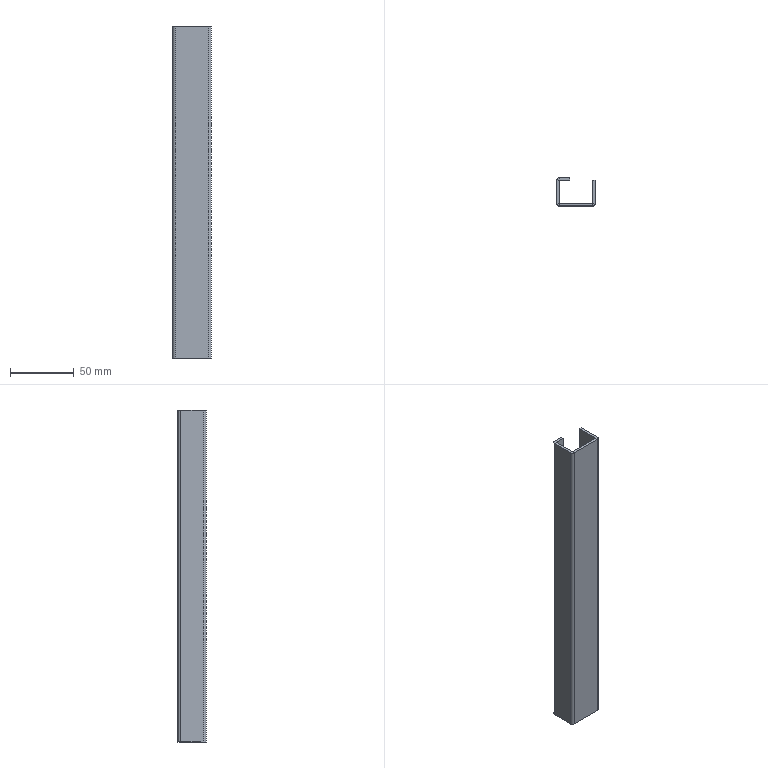Component | SolidWorks | Cover1XG1-2 | 1 solid | 30 faces | box 30 x 22 x 260 mm | volume 38817 mm3 | plane 24 | cylinder 6 | commonest cylinder face diameters 0.1 x3 4.1 x3
STEP:
#1=COLOUR_RGB('',0.7922,0.8196,0.9333);
#2=FILL_AREA_STYLE_COLOUR('',#1);
#3=FILL_AREA_STYLE('',(#2));
#4=SURFACE_STYLE_FILL_AREA(#3);
#5=SURFACE_SIDE_STYLE('',(#4));
#6=SURFACE_STYLE_USAGE(.BOTH.,#5);
#7=PRESENTATION_STYLE_ASSIGNMENT((#6));
#8=CARTESIAN_POINT('',(-5.827,-6.297,10.236));
#9=VERTEX_POINT('',#8);
#10=CARTESIAN_POINT('',(-5.827,-5.593,10.236));
#11=VERTEX_POINT('',#10);
#12=CARTESIAN_POINT('',(-5.827,-6.378,10.236));
#13=DIRECTION('',(0.,1.,0.));
#14=VECTOR('',#13,39.37);
#15=LINE('',#12,#14);
#16=EDGE_CURVE('',#9,#11,#15,.T.);
#17=ORIENTED_EDGE('',*,*,#16,.T.);
#18=CARTESIAN_POINT('',(-5.906,-5.593,10.236));
#19=VERTEX_POINT('',#18);
#20=CARTESIAN_POINT('',(-5.827,-5.593,10.236));
#21=DIRECTION('',(-1.,0.,0.));
#22=VECTOR('',#21,39.37);
#23=LINE('',#20,#22);
#24=EDGE_CURVE('',#11,#19,#23,.T.);
#25=ORIENTED_EDGE('',*,*,#24,.T.);
#26=CARTESIAN_POINT('',(-5.906,-6.297,10.236));
#27=VERTEX_POINT('',#26);
#28=CARTESIAN_POINT('',(-5.906,-6.378,10.236));
#29=DIRECTION('',(0.,1.,0.));
#30=VECTOR('',#29,39.37);
#31=LINE('',#28,#30);
#32=EDGE_CURVE('',#27,#19,#31,.T.);
#33=ORIENTED_EDGE('',*,*,#32,.F.);
#34=CARTESIAN_POINT('',(-5.906,-6.297,10.236));
#35=DIRECTION('',(1.,-0.,0.));
#36=VECTOR('',#35,39.37);
#37=LINE('',#34,#36);
#38=EDGE_CURVE('',#27,#9,#37,.T.);
#39=ORIENTED_EDGE('',*,*,#38,.T.);
#40=EDGE_LOOP('',(#17,#25,#33,#39));
#41=FACE_OUTER_BOUND('',#40,.T.);
#42=CARTESIAN_POINT('',(-5.825,-6.299,10.236));
#43=DIRECTION('',(0.,0.,1.));
#44=DIRECTION('',(-1.,0.,0.));
#45=AXIS2_PLACEMENT_3D('',#42,#43,#44);
#46=PLANE('',#45);
#47=ADVANCED_FACE('',(#41),#46,.T.);
#48=CARTESIAN_POINT('',(-5.906,-5.593,0.));
#49=VERTEX_POINT('',#48);
#50=CARTESIAN_POINT('',(-5.906,-5.593,10.236));
#51=DIRECTION('',(0.,0.,-1.));
#52=VECTOR('',#51,39.37);
#53=LINE('',#50,#52);
#54=EDGE_CURVE('',#19,#49,#53,.T.);
#55=ORIENTED_EDGE('',*,*,#54,.T.);
#56=CARTESIAN_POINT('',(-5.906,-6.297,0.));
#57=VERTEX_POINT('',#56);
#58=CARTESIAN_POINT('',(-5.906,-6.378,0.));
#59=DIRECTION('',(0.,1.,0.));
#60=VECTOR('',#59,39.37);
#61=LINE('',#58,#60);
#62=EDGE_CURVE('',#57,#49,#61,.T.);
#63=ORIENTED_EDGE('',*,*,#62,.F.);
#64=CARTESIAN_POINT('',(-5.906,-6.297,0.));
#65=DIRECTION('',(0.,0.,1.));
#66=VECTOR('',#65,39.37);
#67=LINE('',#64,#66);
#68=EDGE_CURVE('',#57,#27,#67,.T.);
#69=ORIENTED_EDGE('',*,*,#68,.T.);
#70=ORIENTED_EDGE('',*,*,#32,.T.);
#71=EDGE_LOOP('',(#55,#63,#69,#70));
#72=FACE_OUTER_BOUND('',#71,.T.);
#73=CARTESIAN_POINT('',(-5.906,-6.378,0.));
#74=DIRECTION('',(1.,-0.,0.));
#75=DIRECTION('',(-0.,-1.,0.));
#76=AXIS2_PLACEMENT_3D('',#73,#74,#75);
#77=PLANE('',#76);
#78=ADVANCED_FACE('',(#72),#77,.F.);
#79=CARTESIAN_POINT('',(-5.827,-6.297,0.));
#80=VERTEX_POINT('',#79);
#81=CARTESIAN_POINT('',(-5.827,-5.593,0.));
#82=VERTEX_POINT('',#81);
#83=CARTESIAN_POINT('',(-5.827,-6.378,0.));
#84=DIRECTION('',(0.,1.,0.));
#85=VECTOR('',#84,39.37);
#86=LINE('',#83,#85);
#87=EDGE_CURVE('',#80,#82,#86,.T.);
#88=ORIENTED_EDGE('',*,*,#87,.T.);
#89=CARTESIAN_POINT('',(-5.827,-5.593,10.236));
#90=DIRECTION('',(0.,0.,-1.));
#91=VECTOR('',#90,39.37);
#92=LINE('',#89,#91);
#93=EDGE_CURVE('',#11,#82,#92,.T.);
#94=ORIENTED_EDGE('',*,*,#93,.F.);
#95=ORIENTED_EDGE('',*,*,#16,.F.);
#96=CARTESIAN_POINT('',(-5.827,-6.297,0.));
#97=DIRECTION('',(0.,0.,1.));
#98=VECTOR('',#97,39.37);
#99=LINE('',#96,#98);
#100=EDGE_CURVE('',#80,#9,#99,.T.);
#101=ORIENTED_EDGE('',*,*,#100,.F.);
#102=EDGE_LOOP('',(#88,#94,#95,#101));
#103=FACE_OUTER_BOUND('',#102,.T.);
#104=CARTESIAN_POINT('',(-5.827,-6.378,0.));
#105=DIRECTION('',(1.,-0.,0.));
#106=DIRECTION('',(-0.,-1.,0.));
#107=AXIS2_PLACEMENT_3D('',#104,#105,#106);
#108=PLANE('',#107);
#109=ADVANCED_FACE('',(#103),#108,.T.);
#110=CARTESIAN_POINT('',(-4.724,-6.297,0.));
#111=VERTEX_POINT('',#110);
#112=CARTESIAN_POINT('',(-4.803,-6.297,0.));
#113=VERTEX_POINT('',#112);
#114=CARTESIAN_POINT('',(-4.724,-6.297,0.));
#115=DIRECTION('',(-1.,0.,0.));
#116=VECTOR('',#115,39.37);
#117=LINE('',#114,#116);
#118=EDGE_CURVE('',#111,#113,#117,.T.);
#119=ORIENTED_EDGE('',*,*,#118,.F.);
#120=CARTESIAN_POINT('',(-4.805,-6.378,0.));
#121=VERTEX_POINT('',#120);
#122=CARTESIAN_POINT('',(-4.805,-6.297,0.));
#123=DIRECTION('',(0.,0.,-1.));
#124=DIRECTION('',(-1.,0.,0.));
#125=AXIS2_PLACEMENT_3D('',#122,#123,#124);
#126=CIRCLE('',#125,0.08071);
#127=EDGE_CURVE('',#111,#121,#126,.T.);
#128=ORIENTED_EDGE('',*,*,#127,.T.);
#129=CARTESIAN_POINT('',(-4.805,-6.299,0.));
#130=VERTEX_POINT('',#129);
#131=CARTESIAN_POINT('',(-4.805,-6.299,0.));
#132=DIRECTION('',(0.,-1.,0.));
#133=VECTOR('',#132,39.37);
#134=LINE('',#131,#133);
#135=EDGE_CURVE('',#130,#121,#134,.T.);
#136=ORIENTED_EDGE('',*,*,#135,.F.);
#137=CARTESIAN_POINT('',(-4.805,-6.297,0.));
#138=DIRECTION('',(0.,0.,-1.));
#139=DIRECTION('',(1.,0.,0.));
#140=AXIS2_PLACEMENT_3D('',#137,#138,#139);
#141=CIRCLE('',#140,0.001969);
#142=EDGE_CURVE('',#113,#130,#141,.T.);
#143=ORIENTED_EDGE('',*,*,#142,.F.);
#144=EDGE_LOOP('',(#119,#128,#136,#143));
#145=FACE_OUTER_BOUND('',#144,.T.);
#146=CARTESIAN_POINT('',(-4.724,-6.297,0.));
#147=DIRECTION('',(0.,0.,-1.));
#148=DIRECTION('',(1.,0.,0.));
#149=AXIS2_PLACEMENT_3D('',#146,#147,#148);
#150=PLANE('',#149);
#151=ADVANCED_FACE('',(#145),#150,.T.);
#152=CARTESIAN_POINT('',(-4.724,-5.591,0.));
#153=VERTEX_POINT('',#152);
#154=CARTESIAN_POINT('',(-4.724,-6.378,0.));
#155=DIRECTION('',(-0.,-1.,0.));
#156=VECTOR('',#155,39.37);
#157=LINE('',#154,#156);
#158=EDGE_CURVE('',#153,#111,#157,.T.);
#159=ORIENTED_EDGE('',*,*,#158,.T.);
#160=ORIENTED_EDGE('',*,*,#118,.T.);
#161=CARTESIAN_POINT('',(-4.803,-5.591,0.));
#162=VERTEX_POINT('',#161);
#163=CARTESIAN_POINT('',(-4.803,-6.378,0.));
#164=DIRECTION('',(-0.,-1.,0.));
#165=VECTOR('',#164,39.37);
#166=LINE('',#163,#165);
#167=EDGE_CURVE('',#162,#113,#166,.T.);
#168=ORIENTED_EDGE('',*,*,#167,.F.);
#169=CARTESIAN_POINT('',(-4.724,-5.591,0.));
#170=DIRECTION('',(-1.,0.,0.));
#171=VECTOR('',#170,39.37);
#172=LINE('',#169,#171);
#173=EDGE_CURVE('',#153,#162,#172,.T.);
#174=ORIENTED_EDGE('',*,*,#173,.F.);
#175=EDGE_LOOP('',(#159,#160,#168,#174));
#176=FACE_OUTER_BOUND('',#175,.T.);
#177=CARTESIAN_POINT('',(-4.805,-6.299,0.));
#178=DIRECTION('',(0.,0.,-1.));
#179=DIRECTION('',(1.,0.,0.));
#180=AXIS2_PLACEMENT_3D('',#177,#178,#179);
#181=PLANE('',#180);
#182=ADVANCED_FACE('',(#176),#181,.T.);
#183=CARTESIAN_POINT('',(-4.805,-6.378,10.236));
#184=VERTEX_POINT('',#183);
#185=CARTESIAN_POINT('',(-4.805,-6.299,10.236));
#186=VERTEX_POINT('',#185);
#187=CARTESIAN_POINT('',(-4.805,-6.378,10.236));
#188=DIRECTION('',(0.,1.,0.));
#189=VECTOR('',#188,39.37);
#190=LINE('',#187,#189);
#191=EDGE_CURVE('',#184,#186,#190,.T.);
#192=ORIENTED_EDGE('',*,*,#191,.F.);
#193=CARTESIAN_POINT('',(-4.724,-6.297,10.236));
#194=VERTEX_POINT('',#193);
#195=CARTESIAN_POINT('',(-4.805,-6.297,10.236));
#196=DIRECTION('',(0.,0.,-1.));
#197=DIRECTION('',(-1.,0.,0.));
#198=AXIS2_PLACEMENT_3D('',#195,#196,#197);
#199=CIRCLE('',#198,0.08071);
#200=EDGE_CURVE('',#194,#184,#199,.T.);
#201=ORIENTED_EDGE('',*,*,#200,.F.);
#202=CARTESIAN_POINT('',(-4.803,-6.297,10.236));
#203=VERTEX_POINT('',#202);
#204=CARTESIAN_POINT('',(-4.803,-6.297,10.236));
#205=DIRECTION('',(1.,-0.,0.));
#206=VECTOR('',#205,39.37);
#207=LINE('',#204,#206);
#208=EDGE_CURVE('',#203,#194,#207,.T.);
#209=ORIENTED_EDGE('',*,*,#208,.F.);
#210=CARTESIAN_POINT('',(-4.805,-6.297,10.236));
#211=DIRECTION('',(0.,0.,-1.));
#212=DIRECTION('',(1.,0.,0.));
#213=AXIS2_PLACEMENT_3D('',#210,#211,#212);
#214=CIRCLE('',#213,0.001969);
#215=EDGE_CURVE('',#203,#186,#214,.T.);
#216=ORIENTED_EDGE('',*,*,#215,.T.);
#217=EDGE_LOOP('',(#192,#201,#209,#216));
#218=FACE_OUTER_BOUND('',#217,.T.);
#219=CARTESIAN_POINT('',(-4.805,-6.378,10.236));
#220=DIRECTION('',(0.,0.,1.));
#221=DIRECTION('',(-1.,0.,0.));
#222=AXIS2_PLACEMENT_3D('',#219,#220,#221);
#223=PLANE('',#222);
#224=ADVANCED_FACE('',(#218),#223,.T.);
#225=CARTESIAN_POINT('',(-5.825,-6.378,10.236));
#226=VERTEX_POINT('',#225);
#227=CARTESIAN_POINT('',(-5.906,-6.378,10.236));
#228=DIRECTION('',(-1.,0.,0.));
#229=VECTOR('',#228,39.37);
#230=LINE('',#227,#229);
#231=EDGE_CURVE('',#184,#226,#230,.T.);
#232=ORIENTED_EDGE('',*,*,#231,.F.);
#233=ORIENTED_EDGE('',*,*,#191,.T.);
#234=CARTESIAN_POINT('',(-5.825,-6.299,10.236));
#235=VERTEX_POINT('',#234);
#236=CARTESIAN_POINT('',(-5.906,-6.299,10.236));
#237=DIRECTION('',(-1.,0.,0.));
#238=VECTOR('',#237,39.37);
#239=LINE('',#236,#238);
#240=EDGE_CURVE('',#186,#235,#239,.T.);
#241=ORIENTED_EDGE('',*,*,#240,.T.);
#242=CARTESIAN_POINT('',(-5.825,-6.299,10.236));
#243=DIRECTION('',(0.,-1.,0.));
#244=VECTOR('',#243,39.37);
#245=LINE('',#242,#244);
#246=EDGE_CURVE('',#235,#226,#245,.T.);
#247=ORIENTED_EDGE('',*,*,#246,.T.);
#248=EDGE_LOOP('',(#232,#233,#241,#247));
#249=FACE_OUTER_BOUND('',#248,.T.);
#250=CARTESIAN_POINT('',(-4.803,-6.297,10.236));
#251=DIRECTION('',(0.,0.,1.));
#252=DIRECTION('',(-1.,0.,0.));
#253=AXIS2_PLACEMENT_3D('',#250,#251,#252);
#254=PLANE('',#253);
#255=ADVANCED_FACE('',(#249),#254,.T.);
#256=CARTESIAN_POINT('',(-5.825,-6.378,0.));
#257=VERTEX_POINT('',#256);
#258=CARTESIAN_POINT('',(-5.825,-6.299,0.));
#259=VERTEX_POINT('',#258);
#260=CARTESIAN_POINT('',(-5.825,-6.378,0.));
#261=DIRECTION('',(0.,1.,0.));
#262=VECTOR('',#261,39.37);
#263=LINE('',#260,#262);
#264=EDGE_CURVE('',#257,#259,#263,.T.);
#265=ORIENTED_EDGE('',*,*,#264,.F.);
#266=CARTESIAN_POINT('',(-5.825,-6.297,0.));
#267=DIRECTION('',(0.,0.,-1.));
#268=DIRECTION('',(-1.,0.,0.));
#269=AXIS2_PLACEMENT_3D('',#266,#267,#268);
#270=CIRCLE('',#269,0.08071);
#271=EDGE_CURVE('',#257,#57,#270,.T.);
#272=ORIENTED_EDGE('',*,*,#271,.T.);
#273=CARTESIAN_POINT('',(-5.827,-6.297,0.));
#274=DIRECTION('',(-1.,0.,0.));
#275=VECTOR('',#274,39.37);
#276=LINE('',#273,#275);
#277=EDGE_CURVE('',#80,#57,#276,.T.);
#278=ORIENTED_EDGE('',*,*,#277,.F.);
#279=CARTESIAN_POINT('',(-5.825,-6.297,0.));
#280=DIRECTION('',(0.,0.,-1.));
#281=DIRECTION('',(1.,0.,0.));
#282=AXIS2_PLACEMENT_3D('',#279,#280,#281);
#283=CIRCLE('',#282,0.001969);
#284=EDGE_CURVE('',#259,#80,#283,.T.);
#285=ORIENTED_EDGE('',*,*,#284,.F.);
#286=EDGE_LOOP('',(#265,#272,#278,#285));
#287=FACE_OUTER_BOUND('',#286,.T.);
#288=CARTESIAN_POINT('',(-5.825,-6.378,0.));
#289=DIRECTION('',(0.,0.,-1.));
#290=DIRECTION('',(1.,0.,0.));
#291=AXIS2_PLACEMENT_3D('',#288,#289,#290);
#292=PLANE('',#291);
#293=ADVANCED_FACE('',(#287),#292,.T.);
#294=CARTESIAN_POINT('',(-5.906,-6.378,0.));
#295=DIRECTION('',(-1.,0.,0.));
#296=VECTOR('',#295,39.37);
#297=LINE('',#294,#296);
#298=EDGE_CURVE('',#121,#257,#297,.T.);
#299=ORIENTED_EDGE('',*,*,#298,.T.);
#300=ORIENTED_EDGE('',*,*,#264,.T.);
#301=CARTESIAN_POINT('',(-5.906,-6.299,0.));
#302=DIRECTION('',(-1.,0.,0.));
#303=VECTOR('',#302,39.37);
#304=LINE('',#301,#303);
#305=EDGE_CURVE('',#130,#259,#304,.T.);
#306=ORIENTED_EDGE('',*,*,#305,.F.);
#307=ORIENTED_EDGE('',*,*,#135,.T.);
#308=EDGE_LOOP('',(#299,#300,#306,#307));
#309=FACE_OUTER_BOUND('',#308,.T.);
#310=CARTESIAN_POINT('',(-5.827,-6.297,0.));
#311=DIRECTION('',(0.,0.,-1.));
#312=DIRECTION('',(1.,0.,0.));
#313=AXIS2_PLACEMENT_3D('',#310,#311,#312);
#314=PLANE('',#313);
#315=ADVANCED_FACE('',(#309),#314,.T.);
#316=ORIENTED_EDGE('',*,*,#38,.F.);
#317=CARTESIAN_POINT('',(-5.825,-6.297,10.236));
#318=DIRECTION('',(0.,0.,-1.));
#319=DIRECTION('',(-1.,0.,0.));
#320=AXIS2_PLACEMENT_3D('',#317,#318,#319);
#321=CIRCLE('',#320,0.08071);
#322=EDGE_CURVE('',#226,#27,#321,.T.);
#323=ORIENTED_EDGE('',*,*,#322,.F.);
#324=ORIENTED_EDGE('',*,*,#246,.F.);
#325=CARTESIAN_POINT('',(-5.825,-6.297,10.236));
#326=DIRECTION('',(0.,0.,-1.));
#327=DIRECTION('',(1.,0.,0.));
#328=AXIS2_PLACEMENT_3D('',#325,#326,#327);
#329=CIRCLE('',#328,0.001969);
#330=EDGE_CURVE('',#235,#9,#329,.T.);
#331=ORIENTED_EDGE('',*,*,#330,.T.);
#332=EDGE_LOOP('',(#316,#323,#324,#331));
#333=FACE_OUTER_BOUND('',#332,.T.);
#334=CARTESIAN_POINT('',(-5.906,-6.297,10.236));
#335=DIRECTION('',(0.,0.,1.));
#336=DIRECTION('',(-1.,0.,0.));
#337=AXIS2_PLACEMENT_3D('',#334,#335,#336);
#338=PLANE('',#337);
#339=ADVANCED_FACE('',(#333),#338,.T.);
#340=ORIENTED_EDGE('',*,*,#330,.F.);
#341=CARTESIAN_POINT('',(-5.825,-6.299,0.));
#342=DIRECTION('',(0.,0.,1.));
#343=VECTOR('',#342,39.37);
#344=LINE('',#341,#343);
#345=EDGE_CURVE('',#259,#235,#344,.T.);
#346=ORIENTED_EDGE('',*,*,#345,.F.);
#347=ORIENTED_EDGE('',*,*,#284,.T.);
#348=ORIENTED_EDGE('',*,*,#100,.T.);
#349=EDGE_LOOP('',(#340,#346,#347,#348));
#350=FACE_OUTER_BOUND('',#349,.T.);
#351=CARTESIAN_POINT('',(-5.825,-6.297,0.));
#352=DIRECTION('',(0.,0.,1.));
#353=DIRECTION('',(-1.,0.,0.));
#354=AXIS2_PLACEMENT_3D('',#351,#352,#353);
#355=CYLINDRICAL_SURFACE('',#354,0.001969);
#356=ADVANCED_FACE('',(#350),#355,.F.);
#357=ORIENTED_EDGE('',*,*,#240,.F.);
#358=CARTESIAN_POINT('',(-4.805,-6.299,0.));
#359=DIRECTION('',(0.,0.,1.));
#360=VECTOR('',#359,39.37);
#361=LINE('',#358,#360);
#362=EDGE_CURVE('',#130,#186,#361,.T.);
#363=ORIENTED_EDGE('',*,*,#362,.F.);
#364=ORIENTED_EDGE('',*,*,#305,.T.);
#365=ORIENTED_EDGE('',*,*,#345,.T.);
#366=EDGE_LOOP('',(#357,#363,#364,#365));
#367=FACE_OUTER_BOUND('',#366,.T.);
#368=CARTESIAN_POINT('',(-5.906,-6.299,0.));
#369=DIRECTION('',(0.,1.,0.));
#370=DIRECTION('',(0.,0.,1.));
#371=AXIS2_PLACEMENT_3D('',#368,#369,#370);
#372=PLANE('',#371);
#373=ADVANCED_FACE('',(#367),#372,.T.);
#374=ORIENTED_EDGE('',*,*,#215,.F.);
#375=CARTESIAN_POINT('',(-4.803,-6.297,0.));
#376=DIRECTION('',(0.,0.,1.));
#377=VECTOR('',#376,39.37);
#378=LINE('',#375,#377);
#379=EDGE_CURVE('',#113,#203,#378,.T.);
#380=ORIENTED_EDGE('',*,*,#379,.F.);
#381=ORIENTED_EDGE('',*,*,#142,.T.);
#382=ORIENTED_EDGE('',*,*,#362,.T.);
#383=EDGE_LOOP('',(#374,#380,#381,#382));
#384=FACE_OUTER_BOUND('',#383,.T.);
#385=CARTESIAN_POINT('',(-4.805,-6.297,0.));
#386=DIRECTION('',(0.,0.,1.));
#387=DIRECTION('',(-1.,0.,0.));
#388=AXIS2_PLACEMENT_3D('',#385,#386,#387);
#389=CYLINDRICAL_SURFACE('',#388,0.001969);
#390=ADVANCED_FACE('',(#384),#389,.F.);
#391=CARTESIAN_POINT('',(-4.803,-5.591,10.236));
#392=VERTEX_POINT('',#391);
#393=CARTESIAN_POINT('',(-4.803,-6.378,10.236));
#394=DIRECTION('',(-0.,-1.,0.));
#395=VECTOR('',#394,39.37);
#396=LINE('',#393,#395);
#397=EDGE_CURVE('',#392,#203,#396,.T.);
#398=ORIENTED_EDGE('',*,*,#397,.F.);
#399=CARTESIAN_POINT('',(-4.803,-5.591,0.));
#400=DIRECTION('',(0.,0.,1.));
#401=VECTOR('',#400,39.37);
#402=LINE('',#399,#401);
#403=EDGE_CURVE('',#162,#392,#402,.T.);
#404=ORIENTED_EDGE('',*,*,#403,.F.);
#405=ORIENTED_EDGE('',*,*,#167,.T.);
#406=ORIENTED_EDGE('',*,*,#379,.T.);
#407=EDGE_LOOP('',(#398,#404,#405,#406));
#408=FACE_OUTER_BOUND('',#407,.T.);
#409=CARTESIAN_POINT('',(-4.803,-6.378,0.));
#410=DIRECTION('',(-1.,0.,0.));
#411=DIRECTION('',(0.,1.,0.));
#412=AXIS2_PLACEMENT_3D('',#409,#410,#411);
#413=PLANE('',#412);
#414=ADVANCED_FACE('',(#408),#413,.T.);
#415=CARTESIAN_POINT('',(-4.724,-5.591,10.236));
#416=VERTEX_POINT('',#415);
#417=CARTESIAN_POINT('',(-4.724,-5.591,10.236));
#418=DIRECTION('',(-1.,0.,0.));
#419=VECTOR('',#418,39.37);
#420=LINE('',#417,#419);
#421=EDGE_CURVE('',#416,#392,#420,.T.);
#422=ORIENTED_EDGE('',*,*,#421,.F.);
#423=CARTESIAN_POINT('',(-4.724,-5.591,0.));
#424=DIRECTION('',(0.,0.,1.));
#425=VECTOR('',#424,39.37);
#426=LINE('',#423,#425);
#427=EDGE_CURVE('',#153,#416,#426,.T.);
#428=ORIENTED_EDGE('',*,*,#427,.F.);
#429=ORIENTED_EDGE('',*,*,#173,.T.);
#430=ORIENTED_EDGE('',*,*,#403,.T.);
#431=EDGE_LOOP('',(#422,#428,#429,#430));
#432=FACE_OUTER_BOUND('',#431,.T.);
#433=CARTESIAN_POINT('',(-4.724,-5.591,0.));
#434=DIRECTION('',(0.,1.,0.));
#435=DIRECTION('',(0.,0.,1.));
#436=AXIS2_PLACEMENT_3D('',#433,#434,#435);
#437=PLANE('',#436);
#438=ADVANCED_FACE('',(#432),#437,.T.);
#439=CARTESIAN_POINT('',(-4.724,-6.378,10.236));
#440=DIRECTION('',(-0.,-1.,0.));
#441=VECTOR('',#440,39.37);
#442=LINE('',#439,#441);
#443=EDGE_CURVE('',#416,#194,#442,.T.);
#444=ORIENTED_EDGE('',*,*,#443,.T.);
#445=CARTESIAN_POINT('',(-4.724,-6.297,0.));
#446=DIRECTION('',(0.,0.,1.));
#447=VECTOR('',#446,39.37);
#448=LINE('',#445,#447);
#449=EDGE_CURVE('',#111,#194,#448,.T.);
#450=ORIENTED_EDGE('',*,*,#449,.F.);
#451=ORIENTED_EDGE('',*,*,#158,.F.);
#452=ORIENTED_EDGE('',*,*,#427,.T.);
#453=EDGE_LOOP('',(#444,#450,#451,#452));
#454=FACE_OUTER_BOUND('',#453,.T.);
#455=CARTESIAN_POINT('',(-4.724,-6.378,0.));
#456=DIRECTION('',(-1.,0.,0.));
#457=DIRECTION('',(0.,1.,0.));
#458=AXIS2_PLACEMENT_3D('',#455,#456,#457);
#459=PLANE('',#458);
#460=ADVANCED_FACE('',(#454),#459,.F.);
#461=ORIENTED_EDGE('',*,*,#200,.T.);
#462=CARTESIAN_POINT('',(-4.805,-6.378,0.));
#463=DIRECTION('',(0.,0.,1.));
#464=VECTOR('',#463,39.37);
#465=LINE('',#462,#464);
#466=EDGE_CURVE('',#121,#184,#465,.T.);
#467=ORIENTED_EDGE('',*,*,#466,.F.);
#468=ORIENTED_EDGE('',*,*,#127,.F.);
#469=ORIENTED_EDGE('',*,*,#449,.T.);
#470=EDGE_LOOP('',(#461,#467,#468,#469));
#471=FACE_OUTER_BOUND('',#470,.T.);
#472=CARTESIAN_POINT('',(-4.805,-6.297,0.));
#473=DIRECTION('',(0.,0.,1.));
#474=DIRECTION('',(-1.,0.,0.));
#475=AXIS2_PLACEMENT_3D('',#472,#473,#474);
#476=CYLINDRICAL_SURFACE('',#475,0.08071);
#477=ADVANCED_FACE('',(#471),#476,.T.);
#478=ORIENTED_EDGE('',*,*,#231,.T.);
#479=CARTESIAN_POINT('',(-5.825,-6.378,0.));
#480=DIRECTION('',(0.,0.,1.));
#481=VECTOR('',#480,39.37);
#482=LINE('',#479,#481);
#483=EDGE_CURVE('',#257,#226,#482,.T.);
#484=ORIENTED_EDGE('',*,*,#483,.F.);
#485=ORIENTED_EDGE('',*,*,#298,.F.);
#486=ORIENTED_EDGE('',*,*,#466,.T.);
#487=EDGE_LOOP('',(#478,#484,#485,#486));
#488=FACE_OUTER_BOUND('',#487,.T.);
#489=CARTESIAN_POINT('',(-5.906,-6.378,0.));
#490=DIRECTION('',(0.,1.,0.));
#491=DIRECTION('',(0.,0.,1.));
#492=AXIS2_PLACEMENT_3D('',#489,#490,#491);
#493=PLANE('',#492);
#494=ADVANCED_FACE('',(#488),#493,.F.);
#495=ORIENTED_EDGE('',*,*,#322,.T.);
#496=ORIENTED_EDGE('',*,*,#68,.F.);
#497=ORIENTED_EDGE('',*,*,#271,.F.);
#498=ORIENTED_EDGE('',*,*,#483,.T.);
#499=EDGE_LOOP('',(#495,#496,#497,#498));
#500=FACE_OUTER_BOUND('',#499,.T.);
#501=CARTESIAN_POINT('',(-5.825,-6.297,0.));
#502=DIRECTION('',(0.,0.,1.));
#503=DIRECTION('',(-1.,0.,0.));
#504=AXIS2_PLACEMENT_3D('',#501,#502,#503);
#505=CYLINDRICAL_SURFACE('',#504,0.08071);
#506=ADVANCED_FACE('',(#500),#505,.T.);
#507=CARTESIAN_POINT('',(-5.827,-5.593,0.));
#508=DIRECTION('',(-1.,0.,-0.));
#509=VECTOR('',#508,39.37);
#510=LINE('',#507,#509);
#511=EDGE_CURVE('',#82,#49,#510,.T.);
#512=ORIENTED_EDGE('',*,*,#511,.F.);
#513=ORIENTED_EDGE('',*,*,#87,.F.);
#514=ORIENTED_EDGE('',*,*,#277,.T.);
#515=ORIENTED_EDGE('',*,*,#62,.T.);
#516=EDGE_LOOP('',(#512,#513,#514,#515));
#517=FACE_OUTER_BOUND('',#516,.T.);
#518=CARTESIAN_POINT('',(-5.825,-6.297,0.));
#519=DIRECTION('',(0.,0.,-1.));
#520=DIRECTION('',(1.,0.,0.));
#521=AXIS2_PLACEMENT_3D('',#518,#519,#520);
#522=PLANE('',#521);
#523=ADVANCED_FACE('',(#517),#522,.T.);
#524=ORIENTED_EDGE('',*,*,#397,.T.);
#525=ORIENTED_EDGE('',*,*,#208,.T.);
#526=ORIENTED_EDGE('',*,*,#443,.F.);
#527=ORIENTED_EDGE('',*,*,#421,.T.);
#528=EDGE_LOOP('',(#524,#525,#526,#527));
#529=FACE_OUTER_BOUND('',#528,.T.);
#530=CARTESIAN_POINT('',(-5.825,-6.297,10.236));
#531=DIRECTION('',(0.,0.,-1.));
#532=DIRECTION('',(1.,0.,0.));
#533=AXIS2_PLACEMENT_3D('',#530,#531,#532);
#534=PLANE('',#533);
#535=ADVANCED_FACE('',(#529),#534,.F.);
#536=CARTESIAN_POINT('',(-5.825,-5.591,0.));
#537=VERTEX_POINT('',#536);
#538=CARTESIAN_POINT('',(-5.825,-5.512,0.));
#539=VERTEX_POINT('',#538);
#540=CARTESIAN_POINT('',(-5.825,-5.512,0.));
#541=DIRECTION('',(-0.,1.,0.));
#542=VECTOR('',#541,39.37);
#543=LINE('',#540,#542);
#544=EDGE_CURVE('',#537,#539,#543,.T.);
#545=ORIENTED_EDGE('',*,*,#544,.F.);
#546=CARTESIAN_POINT('',(-5.825,-5.593,0.));
#547=DIRECTION('',(0.,0.,-1.));
#548=DIRECTION('',(-1.,0.,0.));
#549=AXIS2_PLACEMENT_3D('',#546,#547,#548);
#550=CIRCLE('',#549,0.001969);
#551=EDGE_CURVE('',#82,#537,#550,.T.);
#552=ORIENTED_EDGE('',*,*,#551,.F.);
#553=ORIENTED_EDGE('',*,*,#511,.T.);
#554=CARTESIAN_POINT('',(-5.825,-5.593,0.));
#555=DIRECTION('',(0.,0.,-1.));
#556=DIRECTION('',(-1.,0.,0.));
#557=AXIS2_PLACEMENT_3D('',#554,#555,#556);
#558=CIRCLE('',#557,0.08071);
#559=EDGE_CURVE('',#49,#539,#558,.T.);
#560=ORIENTED_EDGE('',*,*,#559,.T.);
#561=EDGE_LOOP('',(#545,#552,#553,#560));
#562=FACE_OUTER_BOUND('',#561,.T.);
#563=CARTESIAN_POINT('',(-5.825,-5.593,0.));
#564=DIRECTION('',(0.,0.,-1.));
#565=DIRECTION('',(1.,0.,0.));
#566=AXIS2_PLACEMENT_3D('',#563,#564,#565);
#567=PLANE('',#566);
#568=ADVANCED_FACE('',(#562),#567,.T.);
#569=CARTESIAN_POINT('',(-5.825,-5.591,10.236));
#570=VERTEX_POINT('',#569);
#571=CARTESIAN_POINT('',(-5.825,-5.593,10.236));
#572=DIRECTION('',(0.,0.,1.));
#573=DIRECTION('',(-1.,0.,0.));
#574=AXIS2_PLACEMENT_3D('',#571,#572,#573);
#575=CIRCLE('',#574,0.001969);
#576=EDGE_CURVE('',#570,#11,#575,.T.);
#577=ORIENTED_EDGE('',*,*,#576,.F.);
#578=CARTESIAN_POINT('',(-5.825,-5.512,10.236));
#579=VERTEX_POINT('',#578);
#580=CARTESIAN_POINT('',(-5.825,-5.591,10.236));
#581=DIRECTION('',(-0.,1.,0.));
#582=VECTOR('',#581,39.37);
#583=LINE('',#580,#582);
#584=EDGE_CURVE('',#570,#579,#583,.T.);
#585=ORIENTED_EDGE('',*,*,#584,.T.);
#586=CARTESIAN_POINT('',(-5.825,-5.593,10.236));
#587=DIRECTION('',(0.,0.,1.));
#588=DIRECTION('',(-1.,0.,0.));
#589=AXIS2_PLACEMENT_3D('',#586,#587,#588);
#590=CIRCLE('',#589,0.08071);
#591=EDGE_CURVE('',#579,#19,#590,.T.);
#592=ORIENTED_EDGE('',*,*,#591,.T.);
#593=ORIENTED_EDGE('',*,*,#24,.F.);
#594=EDGE_LOOP('',(#577,#585,#592,#593));
#595=FACE_OUTER_BOUND('',#594,.T.);
#596=CARTESIAN_POINT('',(-5.825,-5.593,10.236));
#597=DIRECTION('',(0.,0.,-1.));
#598=DIRECTION('',(1.,0.,0.));
#599=AXIS2_PLACEMENT_3D('',#596,#597,#598);
#600=PLANE('',#599);
#601=ADVANCED_FACE('',(#595),#600,.F.);
#602=ORIENTED_EDGE('',*,*,#54,.F.);
#603=ORIENTED_EDGE('',*,*,#591,.F.);
#604=CARTESIAN_POINT('',(-5.825,-5.512,10.236));
#605=DIRECTION('',(0.,0.,1.));
#606=VECTOR('',#605,39.37);
#607=LINE('',#604,#606);
#608=EDGE_CURVE('',#539,#579,#607,.T.);
#609=ORIENTED_EDGE('',*,*,#608,.F.);
#610=ORIENTED_EDGE('',*,*,#559,.F.);
#611=EDGE_LOOP('',(#602,#603,#609,#610));
#612=FACE_OUTER_BOUND('',#611,.T.);
#613=CARTESIAN_POINT('',(-5.825,-5.593,10.236));
#614=DIRECTION('',(0.,0.,1.));
#615=DIRECTION('',(0.,1.,0.));
#616=AXIS2_PLACEMENT_3D('',#613,#614,#615);
#617=CYLINDRICAL_SURFACE('',#616,0.08071);
#618=ADVANCED_FACE('',(#612),#617,.T.);
#619=ORIENTED_EDGE('',*,*,#93,.T.);
#620=ORIENTED_EDGE('',*,*,#551,.T.);
#621=CARTESIAN_POINT('',(-5.825,-5.591,0.));
#622=DIRECTION('',(0.,0.,1.));
#623=VECTOR('',#622,39.37);
#624=LINE('',#621,#623);
#625=EDGE_CURVE('',#537,#570,#624,.T.);
#626=ORIENTED_EDGE('',*,*,#625,.T.);
#627=ORIENTED_EDGE('',*,*,#576,.T.);
#628=EDGE_LOOP('',(#619,#620,#626,#627));
#629=FACE_OUTER_BOUND('',#628,.T.);
#630=CARTESIAN_POINT('',(-5.825,-5.593,10.236));
#631=DIRECTION('',(0.,0.,1.));
#632=DIRECTION('',(0.,1.,0.));
#633=AXIS2_PLACEMENT_3D('',#630,#631,#632);
#634=CYLINDRICAL_SURFACE('',#633,0.001969);
#635=ADVANCED_FACE('',(#629),#634,.F.);
#636=CARTESIAN_POINT('',(-5.512,-5.512,10.236));
#637=VERTEX_POINT('',#636);
#638=CARTESIAN_POINT('',(-5.827,-5.512,10.236));
#639=DIRECTION('',(-1.,-0.,0.));
#640=VECTOR('',#639,39.37);
#641=LINE('',#638,#640);
#642=EDGE_CURVE('',#637,#579,#641,.T.);
#643=ORIENTED_EDGE('',*,*,#642,.T.);
#644=ORIENTED_EDGE('',*,*,#584,.F.);
#645=CARTESIAN_POINT('',(-5.512,-5.591,10.236));
#646=VERTEX_POINT('',#645);
#647=CARTESIAN_POINT('',(-5.906,-5.591,10.236));
#648=DIRECTION('',(-1.,-0.,0.));
#649=VECTOR('',#648,39.37);
#650=LINE('',#647,#649);
#651=EDGE_CURVE('',#646,#570,#650,.T.);
#652=ORIENTED_EDGE('',*,*,#651,.F.);
#653=CARTESIAN_POINT('',(-5.512,-5.512,10.236));
#654=DIRECTION('',(0.,-1.,0.));
#655=VECTOR('',#654,39.37);
#656=LINE('',#653,#655);
#657=EDGE_CURVE('',#637,#646,#656,.T.);
#658=ORIENTED_EDGE('',*,*,#657,.F.);
#659=EDGE_LOOP('',(#643,#644,#652,#658));
#660=FACE_OUTER_BOUND('',#659,.T.);
#661=CARTESIAN_POINT('',(-5.827,-5.512,10.236));
#662=DIRECTION('',(0.,0.,1.));
#663=DIRECTION('',(-1.,0.,0.));
#664=AXIS2_PLACEMENT_3D('',#661,#662,#663);
#665=PLANE('',#664);
#666=ADVANCED_FACE('',(#660),#665,.T.);
#667=CARTESIAN_POINT('',(-5.512,-5.591,0.));
#668=VERTEX_POINT('',#667);
#669=CARTESIAN_POINT('',(-5.906,-5.591,0.));
#670=DIRECTION('',(1.,0.,0.));
#671=VECTOR('',#670,39.37);
#672=LINE('',#669,#671);
#673=EDGE_CURVE('',#537,#668,#672,.T.);
#674=ORIENTED_EDGE('',*,*,#673,.F.);
#675=ORIENTED_EDGE('',*,*,#544,.T.);
#676=CARTESIAN_POINT('',(-5.512,-5.512,0.));
#677=VERTEX_POINT('',#676);
#678=CARTESIAN_POINT('',(-5.512,-5.512,0.));
#679=DIRECTION('',(1.,0.,0.));
#680=VECTOR('',#679,39.37);
#681=LINE('',#678,#680);
#682=EDGE_CURVE('',#539,#677,#681,.T.);
#683=ORIENTED_EDGE('',*,*,#682,.T.);
#684=CARTESIAN_POINT('',(-5.512,-5.512,0.));
#685=DIRECTION('',(0.,-1.,0.));
#686=VECTOR('',#685,39.37);
#687=LINE('',#684,#686);
#688=EDGE_CURVE('',#677,#668,#687,.T.);
#689=ORIENTED_EDGE('',*,*,#688,.T.);
#690=EDGE_LOOP('',(#674,#675,#683,#689));
#691=FACE_OUTER_BOUND('',#690,.T.);
#692=CARTESIAN_POINT('',(-5.512,-5.512,0.));
#693=DIRECTION('',(0.,0.,-1.));
#694=DIRECTION('',(1.,0.,0.));
#695=AXIS2_PLACEMENT_3D('',#692,#693,#694);
#696=PLANE('',#695);
#697=ADVANCED_FACE('',(#691),#696,.T.);
#698=ORIENTED_EDGE('',*,*,#682,.F.);
#699=ORIENTED_EDGE('',*,*,#608,.T.);
#700=ORIENTED_EDGE('',*,*,#642,.F.);
#701=CARTESIAN_POINT('',(-5.512,-5.512,10.236));
#702=DIRECTION('',(0.,0.,1.));
#703=VECTOR('',#702,39.37);
#704=LINE('',#701,#703);
#705=EDGE_CURVE('',#677,#637,#704,.T.);
#706=ORIENTED_EDGE('',*,*,#705,.F.);
#707=EDGE_LOOP('',(#698,#699,#700,#706));
#708=FACE_OUTER_BOUND('',#707,.T.);
#709=CARTESIAN_POINT('',(-5.906,-5.512,10.236));
#710=DIRECTION('',(-0.,1.,0.));
#711=DIRECTION('',(1.,0.,0.));
#712=AXIS2_PLACEMENT_3D('',#709,#710,#711);
#713=PLANE('',#712);
#714=ADVANCED_FACE('',(#708),#713,.T.);
#715=ORIENTED_EDGE('',*,*,#625,.F.);
#716=ORIENTED_EDGE('',*,*,#673,.T.);
#717=CARTESIAN_POINT('',(-5.512,-5.591,10.236));
#718=DIRECTION('',(0.,0.,1.));
#719=VECTOR('',#718,39.37);
#720=LINE('',#717,#719);
#721=EDGE_CURVE('',#668,#646,#720,.T.);
#722=ORIENTED_EDGE('',*,*,#721,.T.);
#723=ORIENTED_EDGE('',*,*,#651,.T.);
#724=EDGE_LOOP('',(#715,#716,#722,#723));
#725=FACE_OUTER_BOUND('',#724,.T.);
#726=CARTESIAN_POINT('',(-5.906,-5.591,10.236));
#727=DIRECTION('',(-0.,1.,0.));
#728=DIRECTION('',(1.,0.,0.));
#729=AXIS2_PLACEMENT_3D('',#726,#727,#728);
#730=PLANE('',#729);
#731=ADVANCED_FACE('',(#725),#730,.F.);
#732=ORIENTED_EDGE('',*,*,#721,.F.);
#733=ORIENTED_EDGE('',*,*,#688,.F.);
#734=ORIENTED_EDGE('',*,*,#705,.T.);
#735=ORIENTED_EDGE('',*,*,#657,.T.);
#736=EDGE_LOOP('',(#732,#733,#734,#735));
#737=FACE_OUTER_BOUND('',#736,.T.);
#738=CARTESIAN_POINT('',(-5.512,-5.512,10.236));
#739=DIRECTION('',(1.,0.,0.));
#740=DIRECTION('',(0.,-1.,0.));
#741=AXIS2_PLACEMENT_3D('',#738,#739,#740);
#742=PLANE('',#741);
#743=ADVANCED_FACE('',(#737),#742,.T.);
#744=CLOSED_SHELL('',(#47,#78,#109,#151,#182,#224,#255,#293,#315,#339,#356,#373,#390,#414,#438,#460,#477,#494,#506,#523,#535,#568,#601,#618,#635,#666,#697,#714,#731,#743));
#745=MANIFOLD_SOLID_BREP('',#744);
#746=STYLED_ITEM('',(#7),#745);
#747=PRESENTATION_LAYER_ASSIGNMENT('','',(#746));
#748=CARTESIAN_POINT('',(0.,0.,0.));
#749=DIRECTION('',(0.,0.,1.));
#750=DIRECTION('',(1.,0.,0.));
#751=AXIS2_PLACEMENT_3D('',#748,#749,#750);
#752=(LENGTH_UNIT()NAMED_UNIT(*)SI_UNIT($,.METRE.));
#753=LENGTH_MEASURE_WITH_UNIT(LENGTH_MEASURE(0.0254),#752);
#754=DIMENSIONAL_EXPONENTS(1.,0.,0.,0.,0.,0.,0.);
#755=(CONVERSION_BASED_UNIT('',#753)LENGTH_UNIT()NAMED_UNIT(#754));
#756=UNCERTAINTY_MEASURE_WITH_UNIT(LENGTH_MEASURE(0.00001),#755,'','');
#757=(NAMED_UNIT(*)PLANE_ANGLE_UNIT()SI_UNIT($,.RADIAN.));
#758=(NAMED_UNIT(*)SI_UNIT($,.STERADIAN.)SOLID_ANGLE_UNIT());
#759=(GEOMETRIC_REPRESENTATION_CONTEXT(3)GLOBAL_UNCERTAINTY_ASSIGNED_CONTEXT((#756))GLOBAL_UNIT_ASSIGNED_CONTEXT((#755,#757,#758))REPRESENTATION_CONTEXT('',''));
#760=ADVANCED_BREP_SHAPE_REPRESENTATION('',(#745,#751),#759);
#761=(LENGTH_UNIT()NAMED_UNIT(*)SI_UNIT($,.METRE.));
#762=LENGTH_MEASURE_WITH_UNIT(LENGTH_MEASURE(0.0254),#761);
#763=DIMENSIONAL_EXPONENTS(1.,0.,0.,0.,0.,0.,0.);
#764=(CONVERSION_BASED_UNIT('',#762)LENGTH_UNIT()NAMED_UNIT(#763));
#765=UNCERTAINTY_MEASURE_WITH_UNIT(LENGTH_MEASURE(0.00001),#764,'','');
#766=(NAMED_UNIT(*)PLANE_ANGLE_UNIT()SI_UNIT($,.RADIAN.));
#767=(NAMED_UNIT(*)SI_UNIT($,.STERADIAN.)SOLID_ANGLE_UNIT());
#768=(GEOMETRIC_REPRESENTATION_CONTEXT(3)GLOBAL_UNCERTAINTY_ASSIGNED_CONTEXT((#765))GLOBAL_UNIT_ASSIGNED_CONTEXT((#764,#766,#767))REPRESENTATION_CONTEXT('',''));
#769=MECHANICAL_DESIGN_GEOMETRIC_PRESENTATION_REPRESENTATION('',(#746),#768);